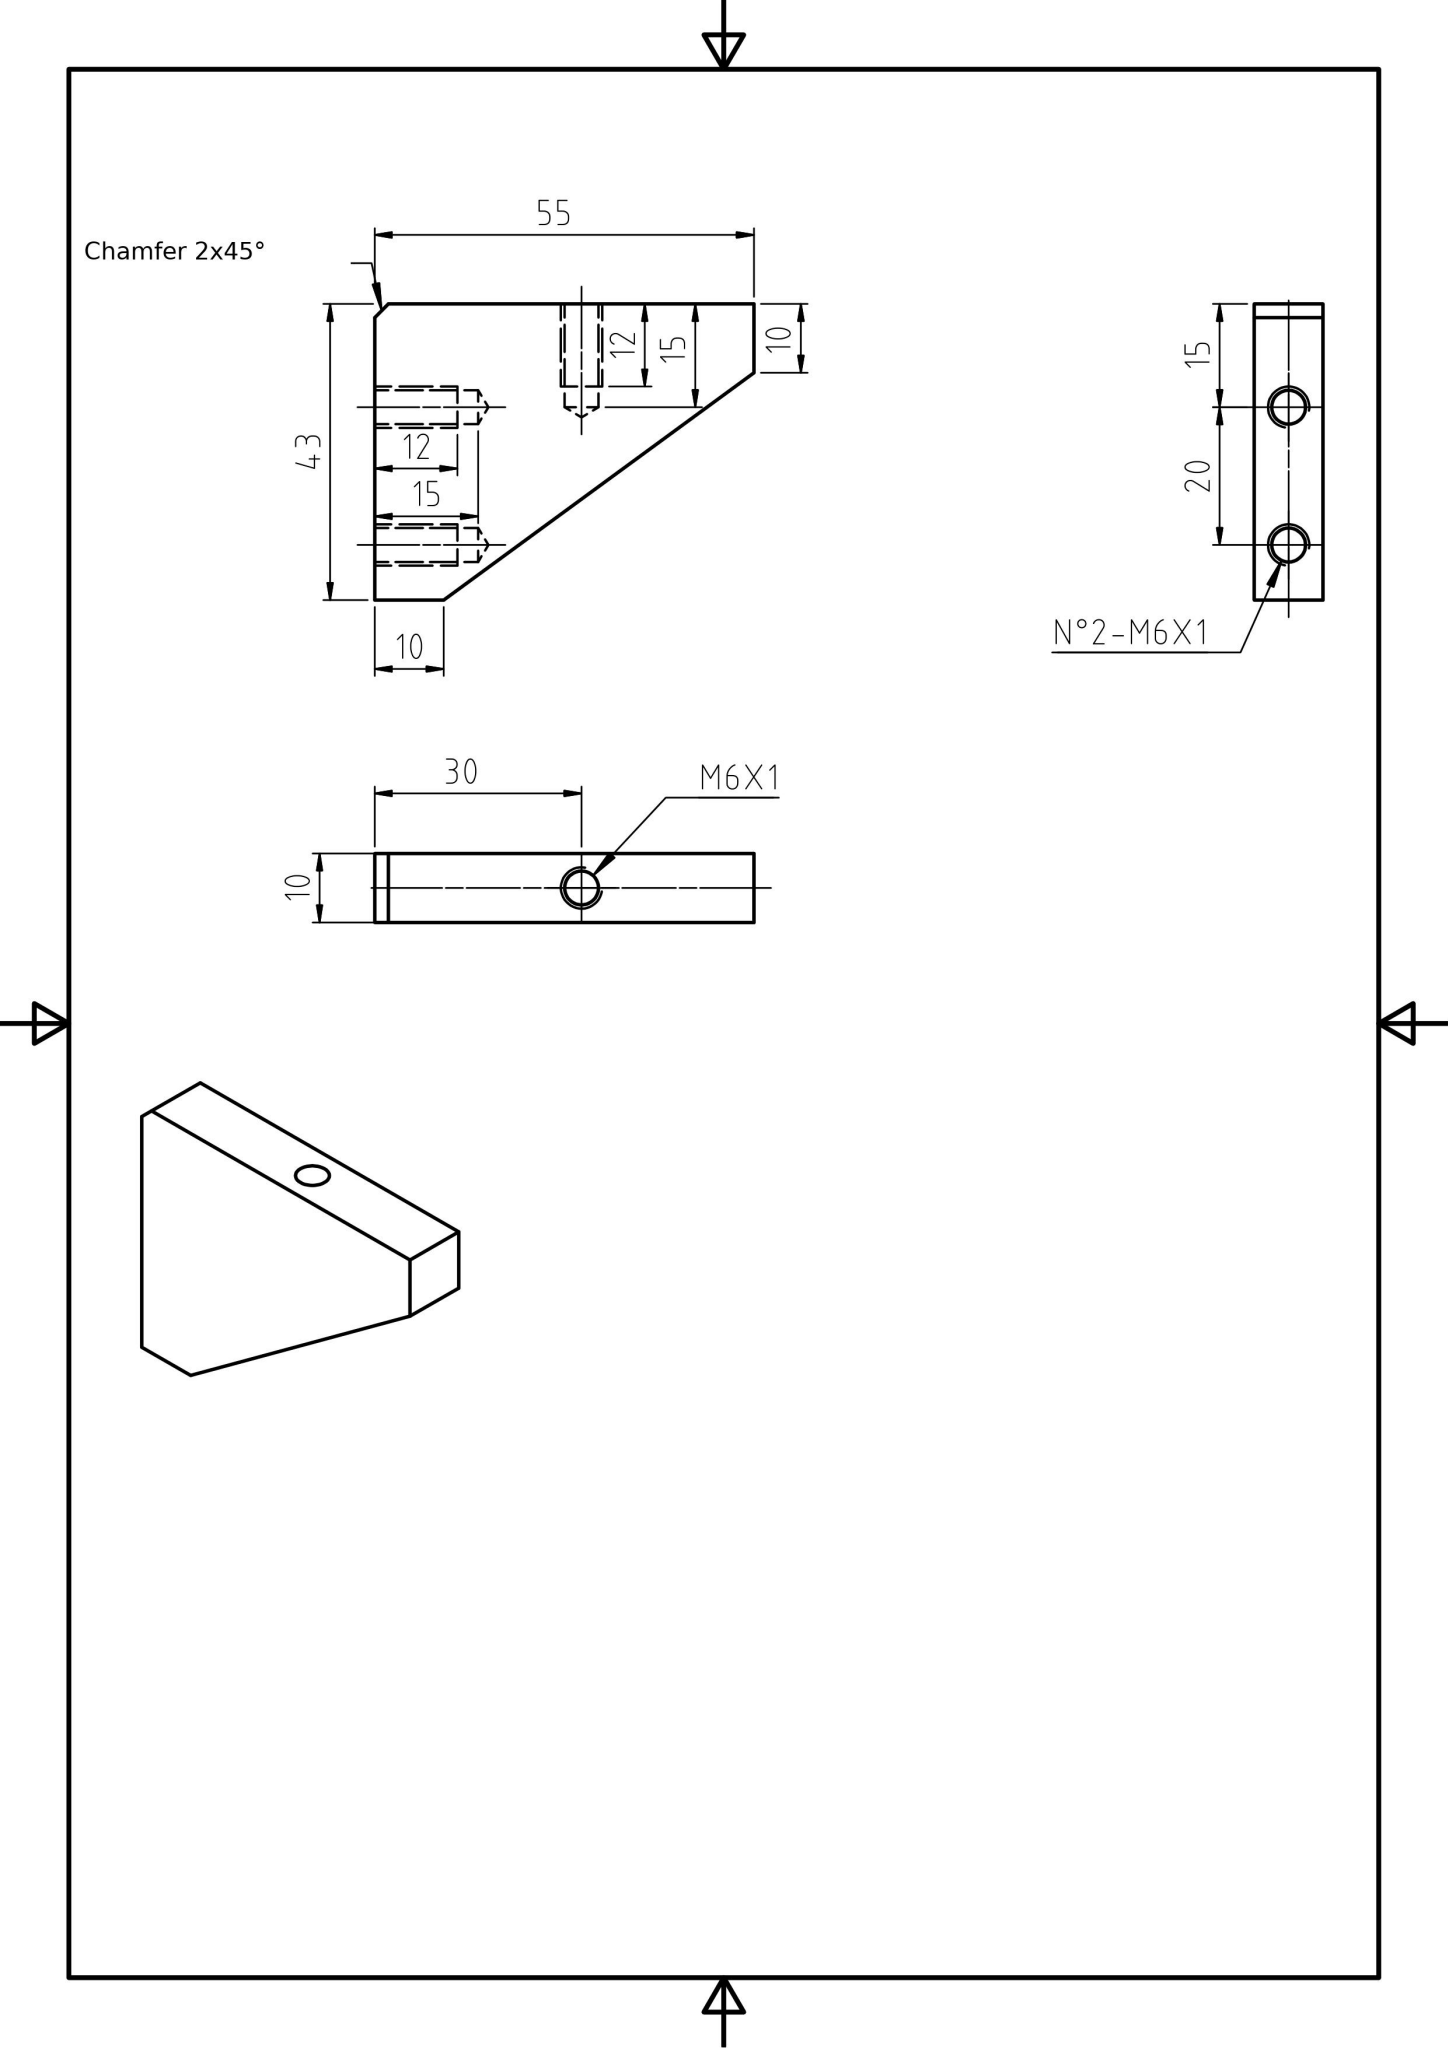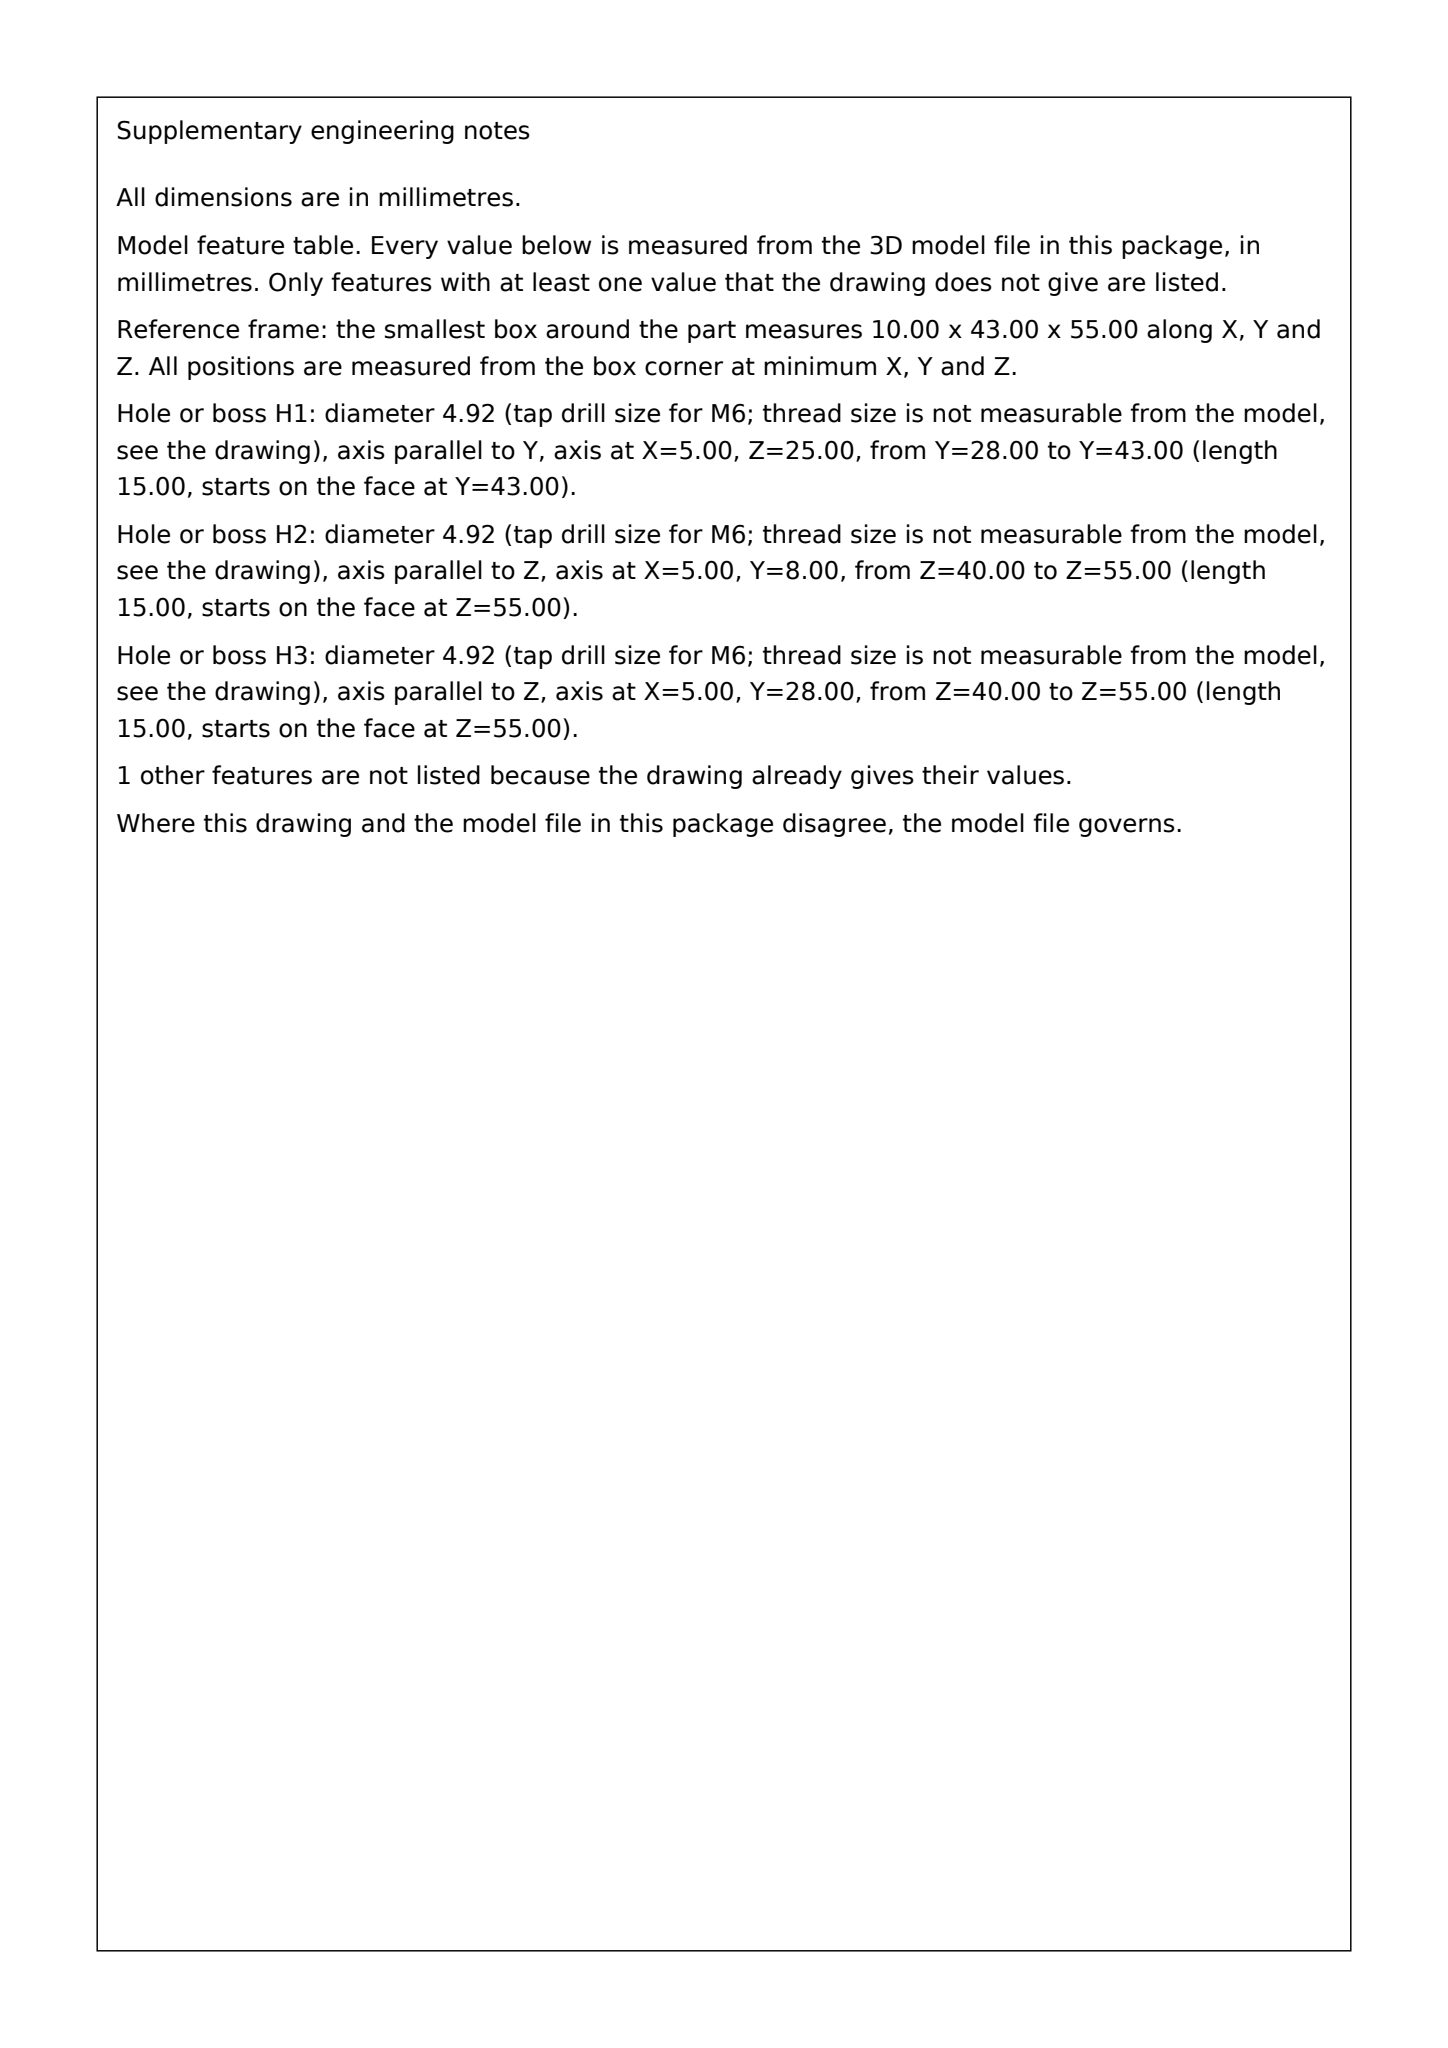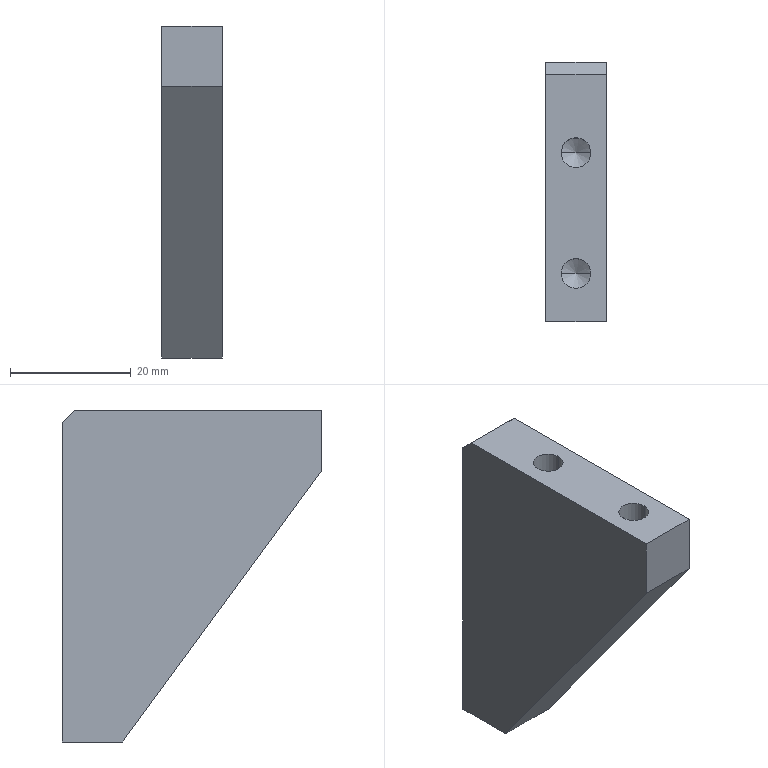Part | SolidWorks | mm | 1 solid | 20 faces | box 10 x 43 x 55 mm | volume 15322 mm3 | plane 8 | cylinder 6 | cone 6 | commonest cylinder face diameters 4.917 x6
STEP:
#1=CARTESIAN_POINT('',(2.542,-15.,-30.));
#2=VERTEX_POINT('',#1);
#3=CARTESIAN_POINT('',(7.458,-15.,-30.));
#4=VERTEX_POINT('',#3);
#5=CARTESIAN_POINT('',(5.,-15.,-30.));
#6=DIRECTION('',(0.,1.,0.));
#7=DIRECTION('',(1.,0.,0.));
#8=AXIS2_PLACEMENT_3D('',#5,#6,#7);
#9=CIRCLE('',#8,2.458);
#10=EDGE_CURVE('',#2,#4,#9,.T.);
#11=ORIENTED_EDGE('',*,*,#10,.F.);
#12=CARTESIAN_POINT('',(2.542,0.,-30.));
#13=VERTEX_POINT('',#12);
#14=CARTESIAN_POINT('',(2.542,-7.5,-30.));
#15=DIRECTION('',(0.,1.,0.));
#16=VECTOR('',#15,1000.);
#17=LINE('',#14,#16);
#18=EDGE_CURVE('',#2,#13,#17,.T.);
#19=ORIENTED_EDGE('',*,*,#18,.T.);
#20=CARTESIAN_POINT('',(7.458,0.,-30.));
#21=VERTEX_POINT('',#20);
#22=CARTESIAN_POINT('',(5.,0.,-30.));
#23=DIRECTION('',(0.,-1.,-0.));
#24=DIRECTION('',(1.,0.,0.));
#25=AXIS2_PLACEMENT_3D('',#22,#23,#24);
#26=CIRCLE('',#25,2.458);
#27=EDGE_CURVE('',#21,#13,#26,.T.);
#28=ORIENTED_EDGE('',*,*,#27,.F.);
#29=CARTESIAN_POINT('',(7.458,-7.5,-30.));
#30=DIRECTION('',(0.,1.,0.));
#31=VECTOR('',#30,1000.);
#32=LINE('',#29,#31);
#33=EDGE_CURVE('',#4,#21,#32,.T.);
#34=ORIENTED_EDGE('',*,*,#33,.F.);
#35=EDGE_LOOP('',(#11,#19,#28,#34));
#36=FACE_OUTER_BOUND('',#35,.T.);
#37=CARTESIAN_POINT('',(5.,-7.5,-30.));
#38=DIRECTION('',(0.,1.,0.));
#39=DIRECTION('',(1.,0.,0.));
#40=AXIS2_PLACEMENT_3D('',#37,#38,#39);
#41=CYLINDRICAL_SURFACE('',#40,2.458);
#42=ADVANCED_FACE('',(#36),#41,.F.);
#43=CARTESIAN_POINT('',(5.,-16.477,-30.));
#44=VERTEX_POINT('',#43);
#45=CARTESIAN_POINT('',(6.229,-15.739,-30.));
#46=DIRECTION('',(0.8572,0.515,0.));
#47=VECTOR('',#46,1000.);
#48=LINE('',#45,#47);
#49=EDGE_CURVE('',#44,#4,#48,.T.);
#50=ORIENTED_EDGE('',*,*,#49,.F.);
#51=CARTESIAN_POINT('',(3.771,-15.739,-30.));
#52=DIRECTION('',(-0.8572,0.515,0.));
#53=VECTOR('',#52,1000.);
#54=LINE('',#51,#53);
#55=EDGE_CURVE('',#44,#2,#54,.T.);
#56=ORIENTED_EDGE('',*,*,#55,.T.);
#57=ORIENTED_EDGE('',*,*,#10,.T.);
#58=EDGE_LOOP('',(#50,#56,#57));
#59=FACE_OUTER_BOUND('',#58,.T.);
#60=CARTESIAN_POINT('',(5.,-15.739,-30.));
#61=DIRECTION('',(0.,1.,0.));
#62=DIRECTION('',(1.,0.,0.));
#63=AXIS2_PLACEMENT_3D('',#60,#61,#62);
#64=CONICAL_SURFACE('',#63,1.229,1.03);
#65=ADVANCED_FACE('',(#59),#64,.F.);
#66=CARTESIAN_POINT('',(2.542,-35.,-15.));
#67=VERTEX_POINT('',#66);
#68=CARTESIAN_POINT('',(7.458,-35.,-15.));
#69=VERTEX_POINT('',#68);
#70=CARTESIAN_POINT('',(5.,-35.,-15.));
#71=DIRECTION('',(0.,-0.,1.));
#72=DIRECTION('',(1.,0.,0.));
#73=AXIS2_PLACEMENT_3D('',#70,#71,#72);
#74=CIRCLE('',#73,2.458);
#75=EDGE_CURVE('',#67,#69,#74,.T.);
#76=ORIENTED_EDGE('',*,*,#75,.F.);
#77=CARTESIAN_POINT('',(2.542,-35.,-0.));
#78=VERTEX_POINT('',#77);
#79=CARTESIAN_POINT('',(2.542,-35.,-7.5));
#80=DIRECTION('',(0.,-0.,1.));
#81=VECTOR('',#80,1000.);
#82=LINE('',#79,#81);
#83=EDGE_CURVE('',#67,#78,#82,.T.);
#84=ORIENTED_EDGE('',*,*,#83,.T.);
#85=CARTESIAN_POINT('',(7.458,-35.,-0.));
#86=VERTEX_POINT('',#85);
#87=CARTESIAN_POINT('',(5.,-35.,-0.));
#88=DIRECTION('',(0.,0.,-1.));
#89=DIRECTION('',(1.,0.,0.));
#90=AXIS2_PLACEMENT_3D('',#87,#88,#89);
#91=CIRCLE('',#90,2.458);
#92=EDGE_CURVE('',#86,#78,#91,.T.);
#93=ORIENTED_EDGE('',*,*,#92,.F.);
#94=CARTESIAN_POINT('',(7.458,-35.,-7.5));
#95=DIRECTION('',(0.,-0.,1.));
#96=VECTOR('',#95,1000.);
#97=LINE('',#94,#96);
#98=EDGE_CURVE('',#69,#86,#97,.T.);
#99=ORIENTED_EDGE('',*,*,#98,.F.);
#100=EDGE_LOOP('',(#76,#84,#93,#99));
#101=FACE_OUTER_BOUND('',#100,.T.);
#102=CARTESIAN_POINT('',(5.,-35.,-7.5));
#103=DIRECTION('',(0.,-0.,1.));
#104=DIRECTION('',(1.,0.,0.));
#105=AXIS2_PLACEMENT_3D('',#102,#103,#104);
#106=CYLINDRICAL_SURFACE('',#105,2.458);
#107=ADVANCED_FACE('',(#101),#106,.F.);
#108=CARTESIAN_POINT('',(5.,-35.,-16.477));
#109=VERTEX_POINT('',#108);
#110=CARTESIAN_POINT('',(6.229,-35.,-15.739));
#111=DIRECTION('',(0.8572,-0.,0.515));
#112=VECTOR('',#111,1000.);
#113=LINE('',#110,#112);
#114=EDGE_CURVE('',#109,#69,#113,.T.);
#115=ORIENTED_EDGE('',*,*,#114,.F.);
#116=CARTESIAN_POINT('',(3.771,-35.,-15.739));
#117=DIRECTION('',(-0.8572,0.,0.515));
#118=VECTOR('',#117,1000.);
#119=LINE('',#116,#118);
#120=EDGE_CURVE('',#109,#67,#119,.T.);
#121=ORIENTED_EDGE('',*,*,#120,.T.);
#122=ORIENTED_EDGE('',*,*,#75,.T.);
#123=EDGE_LOOP('',(#115,#121,#122));
#124=FACE_OUTER_BOUND('',#123,.T.);
#125=CARTESIAN_POINT('',(5.,-35.,-15.739));
#126=DIRECTION('',(0.,-0.,1.));
#127=DIRECTION('',(1.,0.,0.));
#128=AXIS2_PLACEMENT_3D('',#125,#126,#127);
#129=CONICAL_SURFACE('',#128,1.229,1.03);
#130=ADVANCED_FACE('',(#124),#129,.F.);
#131=CARTESIAN_POINT('',(2.542,-15.,-15.));
#132=VERTEX_POINT('',#131);
#133=CARTESIAN_POINT('',(7.458,-15.,-15.));
#134=VERTEX_POINT('',#133);
#135=CARTESIAN_POINT('',(5.,-15.,-15.));
#136=DIRECTION('',(0.,-0.,1.));
#137=DIRECTION('',(1.,0.,0.));
#138=AXIS2_PLACEMENT_3D('',#135,#136,#137);
#139=CIRCLE('',#138,2.458);
#140=EDGE_CURVE('',#132,#134,#139,.T.);
#141=ORIENTED_EDGE('',*,*,#140,.F.);
#142=CARTESIAN_POINT('',(2.542,-15.,-0.));
#143=VERTEX_POINT('',#142);
#144=CARTESIAN_POINT('',(2.542,-15.,-7.5));
#145=DIRECTION('',(0.,-0.,1.));
#146=VECTOR('',#145,1000.);
#147=LINE('',#144,#146);
#148=EDGE_CURVE('',#132,#143,#147,.T.);
#149=ORIENTED_EDGE('',*,*,#148,.T.);
#150=CARTESIAN_POINT('',(7.458,-15.,-0.));
#151=VERTEX_POINT('',#150);
#152=CARTESIAN_POINT('',(5.,-15.,-0.));
#153=DIRECTION('',(0.,0.,-1.));
#154=DIRECTION('',(1.,0.,0.));
#155=AXIS2_PLACEMENT_3D('',#152,#153,#154);
#156=CIRCLE('',#155,2.458);
#157=EDGE_CURVE('',#151,#143,#156,.T.);
#158=ORIENTED_EDGE('',*,*,#157,.F.);
#159=CARTESIAN_POINT('',(7.458,-15.,-7.5));
#160=DIRECTION('',(0.,-0.,1.));
#161=VECTOR('',#160,1000.);
#162=LINE('',#159,#161);
#163=EDGE_CURVE('',#134,#151,#162,.T.);
#164=ORIENTED_EDGE('',*,*,#163,.F.);
#165=EDGE_LOOP('',(#141,#149,#158,#164));
#166=FACE_OUTER_BOUND('',#165,.T.);
#167=CARTESIAN_POINT('',(5.,-15.,-7.5));
#168=DIRECTION('',(0.,-0.,1.));
#169=DIRECTION('',(1.,0.,0.));
#170=AXIS2_PLACEMENT_3D('',#167,#168,#169);
#171=CYLINDRICAL_SURFACE('',#170,2.458);
#172=ADVANCED_FACE('',(#166),#171,.F.);
#173=CARTESIAN_POINT('',(5.,-15.,-16.477));
#174=VERTEX_POINT('',#173);
#175=CARTESIAN_POINT('',(6.229,-15.,-15.739));
#176=DIRECTION('',(0.8572,-0.,0.515));
#177=VECTOR('',#176,1000.);
#178=LINE('',#175,#177);
#179=EDGE_CURVE('',#174,#134,#178,.T.);
#180=ORIENTED_EDGE('',*,*,#179,.F.);
#181=CARTESIAN_POINT('',(3.771,-15.,-15.739));
#182=DIRECTION('',(-0.8572,0.,0.515));
#183=VECTOR('',#182,1000.);
#184=LINE('',#181,#183);
#185=EDGE_CURVE('',#174,#132,#184,.T.);
#186=ORIENTED_EDGE('',*,*,#185,.T.);
#187=ORIENTED_EDGE('',*,*,#140,.T.);
#188=EDGE_LOOP('',(#180,#186,#187));
#189=FACE_OUTER_BOUND('',#188,.T.);
#190=CARTESIAN_POINT('',(5.,-15.,-15.739));
#191=DIRECTION('',(0.,-0.,1.));
#192=DIRECTION('',(1.,0.,0.));
#193=AXIS2_PLACEMENT_3D('',#190,#191,#192);
#194=CONICAL_SURFACE('',#193,1.229,1.03);
#195=ADVANCED_FACE('',(#189),#194,.F.);
#196=CARTESIAN_POINT('',(10.,-2.,-0.));
#197=VERTEX_POINT('',#196);
#198=CARTESIAN_POINT('',(10.,0.,-2.));
#199=VERTEX_POINT('',#198);
#200=CARTESIAN_POINT('',(10.,0.5,-2.5));
#201=DIRECTION('',(0.,0.7071,-0.7071));
#202=VECTOR('',#201,1000.);
#203=LINE('',#200,#202);
#204=EDGE_CURVE('',#197,#199,#203,.T.);
#205=ORIENTED_EDGE('',*,*,#204,.T.);
#206=CARTESIAN_POINT('',(0.,0.,-2.));
#207=VERTEX_POINT('',#206);
#208=CARTESIAN_POINT('',(0.,0.,-2.));
#209=DIRECTION('',(-1.,0.,0.));
#210=VECTOR('',#209,1000.);
#211=LINE('',#208,#210);
#212=EDGE_CURVE('',#199,#207,#211,.T.);
#213=ORIENTED_EDGE('',*,*,#212,.T.);
#214=CARTESIAN_POINT('',(0.,-2.,-0.));
#215=VERTEX_POINT('',#214);
#216=CARTESIAN_POINT('',(0.,0.5,-2.5));
#217=DIRECTION('',(0.,-0.7071,0.7071));
#218=VECTOR('',#217,1000.);
#219=LINE('',#216,#218);
#220=EDGE_CURVE('',#207,#215,#219,.T.);
#221=ORIENTED_EDGE('',*,*,#220,.T.);
#222=CARTESIAN_POINT('',(0.,-2.,-0.));
#223=DIRECTION('',(1.,0.,0.));
#224=VECTOR('',#223,1000.);
#225=LINE('',#222,#224);
#226=EDGE_CURVE('',#215,#197,#225,.T.);
#227=ORIENTED_EDGE('',*,*,#226,.T.);
#228=EDGE_LOOP('',(#205,#213,#221,#227));
#229=FACE_OUTER_BOUND('',#228,.T.);
#230=CARTESIAN_POINT('',(0.,-1.,-1.));
#231=DIRECTION('',(0.,0.7071,0.7071));
#232=DIRECTION('',(1.,0.,0.));
#233=AXIS2_PLACEMENT_3D('',#230,#231,#232);
#234=PLANE('',#233);
#235=ADVANCED_FACE('',(#229),#234,.T.);
#236=ORIENTED_EDGE('',*,*,#220,.F.);
#237=CARTESIAN_POINT('',(0.,0.,-55.));
#238=VERTEX_POINT('',#237);
#239=CARTESIAN_POINT('',(0.,0.,-55.));
#240=DIRECTION('',(0.,-0.,1.));
#241=VECTOR('',#240,1000.);
#242=LINE('',#239,#241);
#243=EDGE_CURVE('',#238,#207,#242,.T.);
#244=ORIENTED_EDGE('',*,*,#243,.F.);
#245=CARTESIAN_POINT('',(0.,-10.,-55.));
#246=VERTEX_POINT('',#245);
#247=CARTESIAN_POINT('',(0.,-43.,-55.));
#248=DIRECTION('',(0.,1.,0.));
#249=VECTOR('',#248,1000.);
#250=LINE('',#247,#249);
#251=EDGE_CURVE('',#246,#238,#250,.T.);
#252=ORIENTED_EDGE('',*,*,#251,.F.);
#253=CARTESIAN_POINT('',(0.,-43.,-10.));
#254=VERTEX_POINT('',#253);
#255=CARTESIAN_POINT('',(0.,-43.,-10.));
#256=DIRECTION('',(0.,0.5914,-0.8064));
#257=VECTOR('',#256,1000.);
#258=LINE('',#255,#257);
#259=EDGE_CURVE('',#254,#246,#258,.T.);
#260=ORIENTED_EDGE('',*,*,#259,.F.);
#261=CARTESIAN_POINT('',(0.,-43.,-0.));
#262=VERTEX_POINT('',#261);
#263=CARTESIAN_POINT('',(0.,-43.,-0.));
#264=DIRECTION('',(0.,0.,-1.));
#265=VECTOR('',#264,1000.);
#266=LINE('',#263,#265);
#267=EDGE_CURVE('',#262,#254,#266,.T.);
#268=ORIENTED_EDGE('',*,*,#267,.F.);
#269=CARTESIAN_POINT('',(0.,0.,0.));
#270=DIRECTION('',(0.,-1.,-0.));
#271=VECTOR('',#270,1000.);
#272=LINE('',#269,#271);
#273=EDGE_CURVE('',#215,#262,#272,.T.);
#274=ORIENTED_EDGE('',*,*,#273,.F.);
#275=EDGE_LOOP('',(#236,#244,#252,#260,#268,#274));
#276=FACE_OUTER_BOUND('',#275,.T.);
#277=CARTESIAN_POINT('',(0.,-21.5,-27.5));
#278=DIRECTION('',(1.,0.,0.));
#279=DIRECTION('',(0.,1.,0.));
#280=AXIS2_PLACEMENT_3D('',#277,#278,#279);
#281=PLANE('',#280);
#282=ADVANCED_FACE('',(#276),#281,.F.);
#283=ORIENTED_EDGE('',*,*,#212,.F.);
#284=CARTESIAN_POINT('',(10.,0.,-55.));
#285=VERTEX_POINT('',#284);
#286=CARTESIAN_POINT('',(10.,0.,-55.));
#287=DIRECTION('',(0.,-0.,1.));
#288=VECTOR('',#287,1000.);
#289=LINE('',#286,#288);
#290=EDGE_CURVE('',#285,#199,#289,.T.);
#291=ORIENTED_EDGE('',*,*,#290,.F.);
#292=CARTESIAN_POINT('',(0.,0.,-55.));
#293=DIRECTION('',(1.,0.,0.));
#294=VECTOR('',#293,1000.);
#295=LINE('',#292,#294);
#296=EDGE_CURVE('',#238,#285,#295,.T.);
#297=ORIENTED_EDGE('',*,*,#296,.F.);
#298=ORIENTED_EDGE('',*,*,#243,.T.);
#299=EDGE_LOOP('',(#283,#291,#297,#298));
#300=FACE_OUTER_BOUND('',#299,.T.);
#301=ORIENTED_EDGE('',*,*,#27,.T.);
#302=CARTESIAN_POINT('',(5.,0.,-30.));
#303=DIRECTION('',(0.,-1.,-0.));
#304=DIRECTION('',(1.,0.,0.));
#305=AXIS2_PLACEMENT_3D('',#302,#303,#304);
#306=CIRCLE('',#305,2.458);
#307=EDGE_CURVE('',#13,#21,#306,.T.);
#308=ORIENTED_EDGE('',*,*,#307,.T.);
#309=EDGE_LOOP('',(#301,#308));
#310=FACE_BOUND('',#309,.T.);
#311=CARTESIAN_POINT('',(0.,0.,-55.));
#312=DIRECTION('',(0.,1.,0.));
#313=DIRECTION('',(1.,0.,0.));
#314=AXIS2_PLACEMENT_3D('',#311,#312,#313);
#315=PLANE('',#314);
#316=ADVANCED_FACE('',(#300,#310),#315,.T.);
#317=ORIENTED_EDGE('',*,*,#185,.F.);
#318=ORIENTED_EDGE('',*,*,#179,.T.);
#319=CARTESIAN_POINT('',(5.,-15.,-15.));
#320=DIRECTION('',(0.,-0.,1.));
#321=DIRECTION('',(1.,0.,0.));
#322=AXIS2_PLACEMENT_3D('',#319,#320,#321);
#323=CIRCLE('',#322,2.458);
#324=EDGE_CURVE('',#134,#132,#323,.T.);
#325=ORIENTED_EDGE('',*,*,#324,.T.);
#326=EDGE_LOOP('',(#317,#318,#325));
#327=FACE_OUTER_BOUND('',#326,.T.);
#328=CARTESIAN_POINT('',(5.,-15.,-15.739));
#329=DIRECTION('',(0.,-0.,1.));
#330=DIRECTION('',(1.,0.,0.));
#331=AXIS2_PLACEMENT_3D('',#328,#329,#330);
#332=CONICAL_SURFACE('',#331,1.229,1.03);
#333=ADVANCED_FACE('',(#327),#332,.F.);
#334=ORIENTED_EDGE('',*,*,#148,.F.);
#335=ORIENTED_EDGE('',*,*,#324,.F.);
#336=ORIENTED_EDGE('',*,*,#163,.T.);
#337=CARTESIAN_POINT('',(5.,-15.,-0.));
#338=DIRECTION('',(0.,0.,-1.));
#339=DIRECTION('',(1.,0.,0.));
#340=AXIS2_PLACEMENT_3D('',#337,#338,#339);
#341=CIRCLE('',#340,2.458);
#342=EDGE_CURVE('',#143,#151,#341,.T.);
#343=ORIENTED_EDGE('',*,*,#342,.F.);
#344=EDGE_LOOP('',(#334,#335,#336,#343));
#345=FACE_OUTER_BOUND('',#344,.T.);
#346=CARTESIAN_POINT('',(5.,-15.,-7.5));
#347=DIRECTION('',(0.,-0.,1.));
#348=DIRECTION('',(1.,0.,0.));
#349=AXIS2_PLACEMENT_3D('',#346,#347,#348);
#350=CYLINDRICAL_SURFACE('',#349,2.458);
#351=ADVANCED_FACE('',(#345),#350,.F.);
#352=ORIENTED_EDGE('',*,*,#120,.F.);
#353=ORIENTED_EDGE('',*,*,#114,.T.);
#354=CARTESIAN_POINT('',(5.,-35.,-15.));
#355=DIRECTION('',(0.,-0.,1.));
#356=DIRECTION('',(1.,0.,0.));
#357=AXIS2_PLACEMENT_3D('',#354,#355,#356);
#358=CIRCLE('',#357,2.458);
#359=EDGE_CURVE('',#69,#67,#358,.T.);
#360=ORIENTED_EDGE('',*,*,#359,.T.);
#361=EDGE_LOOP('',(#352,#353,#360));
#362=FACE_OUTER_BOUND('',#361,.T.);
#363=CARTESIAN_POINT('',(5.,-35.,-15.739));
#364=DIRECTION('',(0.,-0.,1.));
#365=DIRECTION('',(1.,0.,0.));
#366=AXIS2_PLACEMENT_3D('',#363,#364,#365);
#367=CONICAL_SURFACE('',#366,1.229,1.03);
#368=ADVANCED_FACE('',(#362),#367,.F.);
#369=ORIENTED_EDGE('',*,*,#83,.F.);
#370=ORIENTED_EDGE('',*,*,#359,.F.);
#371=ORIENTED_EDGE('',*,*,#98,.T.);
#372=CARTESIAN_POINT('',(5.,-35.,-0.));
#373=DIRECTION('',(0.,0.,-1.));
#374=DIRECTION('',(1.,0.,0.));
#375=AXIS2_PLACEMENT_3D('',#372,#373,#374);
#376=CIRCLE('',#375,2.458);
#377=EDGE_CURVE('',#78,#86,#376,.T.);
#378=ORIENTED_EDGE('',*,*,#377,.F.);
#379=EDGE_LOOP('',(#369,#370,#371,#378));
#380=FACE_OUTER_BOUND('',#379,.T.);
#381=CARTESIAN_POINT('',(5.,-35.,-7.5));
#382=DIRECTION('',(0.,-0.,1.));
#383=DIRECTION('',(1.,0.,0.));
#384=AXIS2_PLACEMENT_3D('',#381,#382,#383);
#385=CYLINDRICAL_SURFACE('',#384,2.458);
#386=ADVANCED_FACE('',(#380),#385,.F.);
#387=ORIENTED_EDGE('',*,*,#55,.F.);
#388=ORIENTED_EDGE('',*,*,#49,.T.);
#389=CARTESIAN_POINT('',(5.,-15.,-30.));
#390=DIRECTION('',(0.,1.,0.));
#391=DIRECTION('',(1.,0.,0.));
#392=AXIS2_PLACEMENT_3D('',#389,#390,#391);
#393=CIRCLE('',#392,2.458);
#394=EDGE_CURVE('',#4,#2,#393,.T.);
#395=ORIENTED_EDGE('',*,*,#394,.T.);
#396=EDGE_LOOP('',(#387,#388,#395));
#397=FACE_OUTER_BOUND('',#396,.T.);
#398=CARTESIAN_POINT('',(5.,-15.739,-30.));
#399=DIRECTION('',(0.,1.,0.));
#400=DIRECTION('',(1.,0.,0.));
#401=AXIS2_PLACEMENT_3D('',#398,#399,#400);
#402=CONICAL_SURFACE('',#401,1.229,1.03);
#403=ADVANCED_FACE('',(#397),#402,.F.);
#404=ORIENTED_EDGE('',*,*,#18,.F.);
#405=ORIENTED_EDGE('',*,*,#394,.F.);
#406=ORIENTED_EDGE('',*,*,#33,.T.);
#407=ORIENTED_EDGE('',*,*,#307,.F.);
#408=EDGE_LOOP('',(#404,#405,#406,#407));
#409=FACE_OUTER_BOUND('',#408,.T.);
#410=CARTESIAN_POINT('',(5.,-7.5,-30.));
#411=DIRECTION('',(0.,1.,0.));
#412=DIRECTION('',(1.,0.,0.));
#413=AXIS2_PLACEMENT_3D('',#410,#411,#412);
#414=CYLINDRICAL_SURFACE('',#413,2.458);
#415=ADVANCED_FACE('',(#409),#414,.F.);
#416=ORIENTED_EDGE('',*,*,#226,.F.);
#417=ORIENTED_EDGE('',*,*,#273,.T.);
#418=CARTESIAN_POINT('',(10.,-43.,-0.));
#419=VERTEX_POINT('',#418);
#420=CARTESIAN_POINT('',(0.,-43.,-0.));
#421=DIRECTION('',(1.,0.,0.));
#422=VECTOR('',#421,1000.);
#423=LINE('',#420,#422);
#424=EDGE_CURVE('',#262,#419,#423,.T.);
#425=ORIENTED_EDGE('',*,*,#424,.T.);
#426=CARTESIAN_POINT('',(10.,0.,0.));
#427=DIRECTION('',(0.,-1.,-0.));
#428=VECTOR('',#427,1000.);
#429=LINE('',#426,#428);
#430=EDGE_CURVE('',#197,#419,#429,.T.);
#431=ORIENTED_EDGE('',*,*,#430,.F.);
#432=EDGE_LOOP('',(#416,#417,#425,#431));
#433=FACE_OUTER_BOUND('',#432,.T.);
#434=ORIENTED_EDGE('',*,*,#157,.T.);
#435=ORIENTED_EDGE('',*,*,#342,.T.);
#436=EDGE_LOOP('',(#434,#435));
#437=FACE_BOUND('',#436,.T.);
#438=ORIENTED_EDGE('',*,*,#92,.T.);
#439=ORIENTED_EDGE('',*,*,#377,.T.);
#440=EDGE_LOOP('',(#438,#439));
#441=FACE_BOUND('',#440,.T.);
#442=CARTESIAN_POINT('',(0.,0.,0.));
#443=DIRECTION('',(0.,-0.,1.));
#444=DIRECTION('',(1.,0.,0.));
#445=AXIS2_PLACEMENT_3D('',#442,#443,#444);
#446=PLANE('',#445);
#447=ADVANCED_FACE('',(#433,#437,#441),#446,.T.);
#448=ORIENTED_EDGE('',*,*,#251,.T.);
#449=ORIENTED_EDGE('',*,*,#296,.T.);
#450=CARTESIAN_POINT('',(10.,-10.,-55.));
#451=VERTEX_POINT('',#450);
#452=CARTESIAN_POINT('',(10.,-43.,-55.));
#453=DIRECTION('',(0.,1.,0.));
#454=VECTOR('',#453,1000.);
#455=LINE('',#452,#454);
#456=EDGE_CURVE('',#451,#285,#455,.T.);
#457=ORIENTED_EDGE('',*,*,#456,.F.);
#458=CARTESIAN_POINT('',(0.,-10.,-55.));
#459=DIRECTION('',(1.,0.,0.));
#460=VECTOR('',#459,1000.);
#461=LINE('',#458,#460);
#462=EDGE_CURVE('',#246,#451,#461,.T.);
#463=ORIENTED_EDGE('',*,*,#462,.F.);
#464=EDGE_LOOP('',(#448,#449,#457,#463));
#465=FACE_OUTER_BOUND('',#464,.T.);
#466=CARTESIAN_POINT('',(0.,-10.,-55.));
#467=DIRECTION('',(0.,0.,-1.));
#468=DIRECTION('',(-1.,0.,0.));
#469=AXIS2_PLACEMENT_3D('',#466,#467,#468);
#470=PLANE('',#469);
#471=ADVANCED_FACE('',(#465),#470,.T.);
#472=ORIENTED_EDGE('',*,*,#259,.T.);
#473=ORIENTED_EDGE('',*,*,#462,.T.);
#474=CARTESIAN_POINT('',(10.,-43.,-10.));
#475=VERTEX_POINT('',#474);
#476=CARTESIAN_POINT('',(10.,-43.,-10.));
#477=DIRECTION('',(0.,0.5914,-0.8064));
#478=VECTOR('',#477,1000.);
#479=LINE('',#476,#478);
#480=EDGE_CURVE('',#475,#451,#479,.T.);
#481=ORIENTED_EDGE('',*,*,#480,.F.);
#482=CARTESIAN_POINT('',(0.,-43.,-10.));
#483=DIRECTION('',(1.,0.,0.));
#484=VECTOR('',#483,1000.);
#485=LINE('',#482,#484);
#486=EDGE_CURVE('',#254,#475,#485,.T.);
#487=ORIENTED_EDGE('',*,*,#486,.F.);
#488=EDGE_LOOP('',(#472,#473,#481,#487));
#489=FACE_OUTER_BOUND('',#488,.T.);
#490=CARTESIAN_POINT('',(0.,-43.,-10.));
#491=DIRECTION('',(0.,-0.8064,-0.5914));
#492=DIRECTION('',(0.,0.5914,-0.8064));
#493=AXIS2_PLACEMENT_3D('',#490,#491,#492);
#494=PLANE('',#493);
#495=ADVANCED_FACE('',(#489),#494,.T.);
#496=ORIENTED_EDGE('',*,*,#267,.T.);
#497=ORIENTED_EDGE('',*,*,#486,.T.);
#498=CARTESIAN_POINT('',(10.,-43.,-0.));
#499=DIRECTION('',(0.,0.,-1.));
#500=VECTOR('',#499,1000.);
#501=LINE('',#498,#500);
#502=EDGE_CURVE('',#419,#475,#501,.T.);
#503=ORIENTED_EDGE('',*,*,#502,.F.);
#504=ORIENTED_EDGE('',*,*,#424,.F.);
#505=EDGE_LOOP('',(#496,#497,#503,#504));
#506=FACE_OUTER_BOUND('',#505,.T.);
#507=CARTESIAN_POINT('',(0.,-43.,-0.));
#508=DIRECTION('',(0.,-1.,-0.));
#509=DIRECTION('',(0.,0.,-1.));
#510=AXIS2_PLACEMENT_3D('',#507,#508,#509);
#511=PLANE('',#510);
#512=ADVANCED_FACE('',(#506),#511,.T.);
#513=ORIENTED_EDGE('',*,*,#204,.F.);
#514=ORIENTED_EDGE('',*,*,#430,.T.);
#515=ORIENTED_EDGE('',*,*,#502,.T.);
#516=ORIENTED_EDGE('',*,*,#480,.T.);
#517=ORIENTED_EDGE('',*,*,#456,.T.);
#518=ORIENTED_EDGE('',*,*,#290,.T.);
#519=EDGE_LOOP('',(#513,#514,#515,#516,#517,#518));
#520=FACE_OUTER_BOUND('',#519,.T.);
#521=CARTESIAN_POINT('',(10.,-21.5,-27.5));
#522=DIRECTION('',(1.,0.,0.));
#523=DIRECTION('',(0.,1.,0.));
#524=AXIS2_PLACEMENT_3D('',#521,#522,#523);
#525=PLANE('',#524);
#526=ADVANCED_FACE('',(#520),#525,.T.);
#527=CLOSED_SHELL('',(#42,#65,#107,#130,#172,#195,#235,#282,#316,#333,#351,#368,#386,#403,#415,#447,#471,#495,#512,#526));
#528=MANIFOLD_SOLID_BREP('',#527);
#529=CARTESIAN_POINT('',(0.,0.,0.));
#530=DIRECTION('',(0.,0.,1.));
#531=DIRECTION('',(1.,0.,0.));
#532=AXIS2_PLACEMENT_3D('',#529,#530,#531);
#533=(LENGTH_UNIT()NAMED_UNIT(*)SI_UNIT(.MILLI.,.METRE.));
#534=UNCERTAINTY_MEASURE_WITH_UNIT(LENGTH_MEASURE(0.00001),#533,'','');
#535=(NAMED_UNIT(*)PLANE_ANGLE_UNIT()SI_UNIT($,.RADIAN.));
#536=(NAMED_UNIT(*)SI_UNIT($,.STERADIAN.)SOLID_ANGLE_UNIT());
#537=(GEOMETRIC_REPRESENTATION_CONTEXT(3)GLOBAL_UNCERTAINTY_ASSIGNED_CONTEXT((#534))GLOBAL_UNIT_ASSIGNED_CONTEXT((#533,#535,#536))REPRESENTATION_CONTEXT('',''));
#538=ADVANCED_BREP_SHAPE_REPRESENTATION('',(#528,#532),#537);